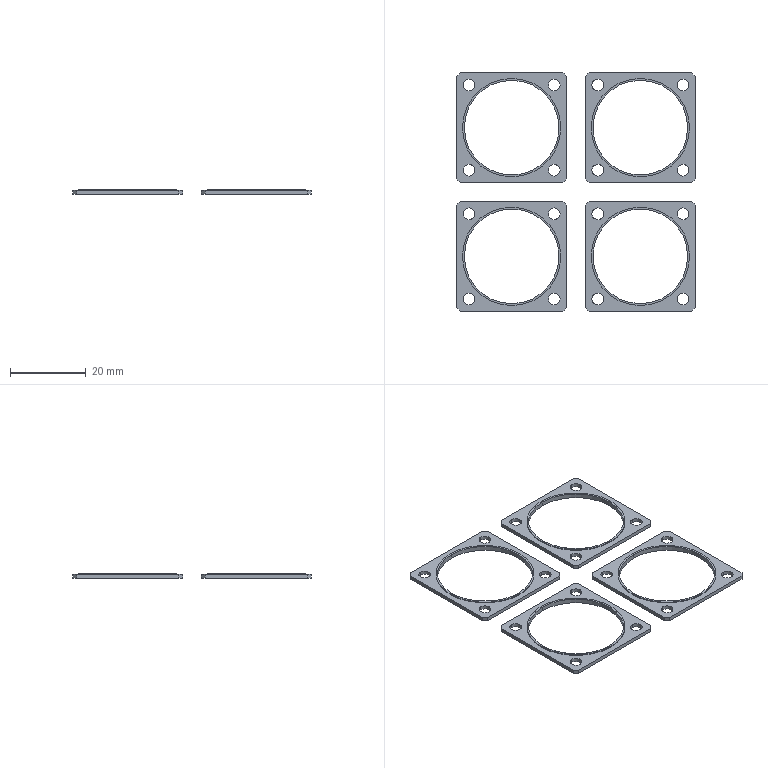CAM job | Mastercam | mm | 9 operations | part box 63 x 63 x 1.2
1. 2D High Speed (2D Area Mill) | 1 - 6C
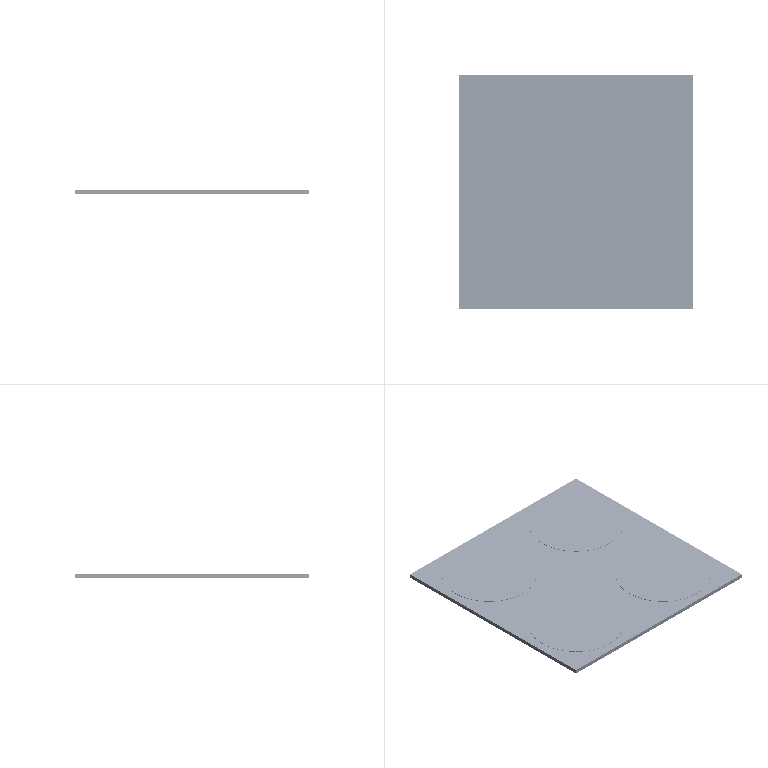2. Contour (Ramp) | 1 - 6C
3. Contour (Ramp) | 3 - 2C
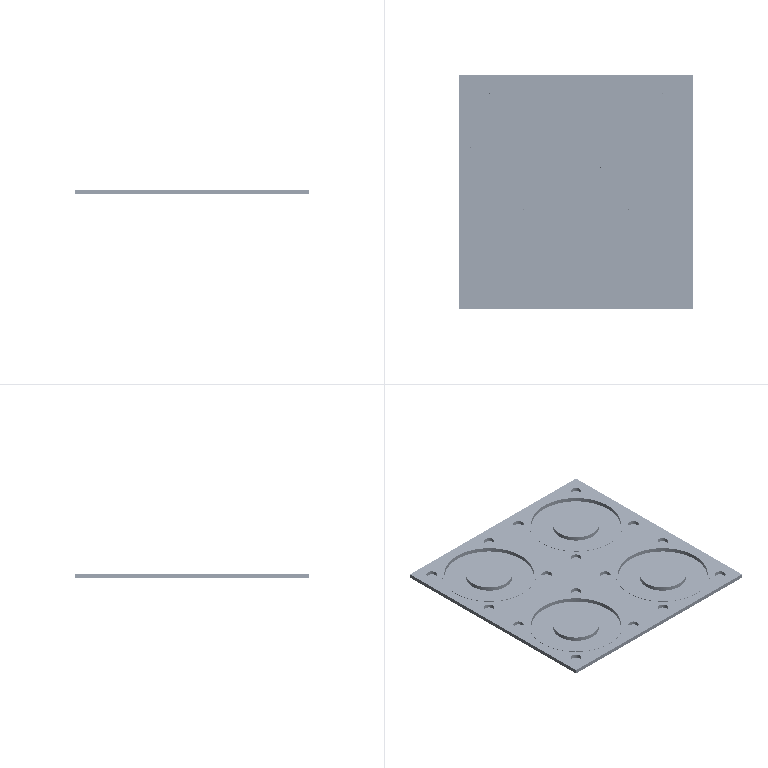4. Contour (2D) | 4 - 2J
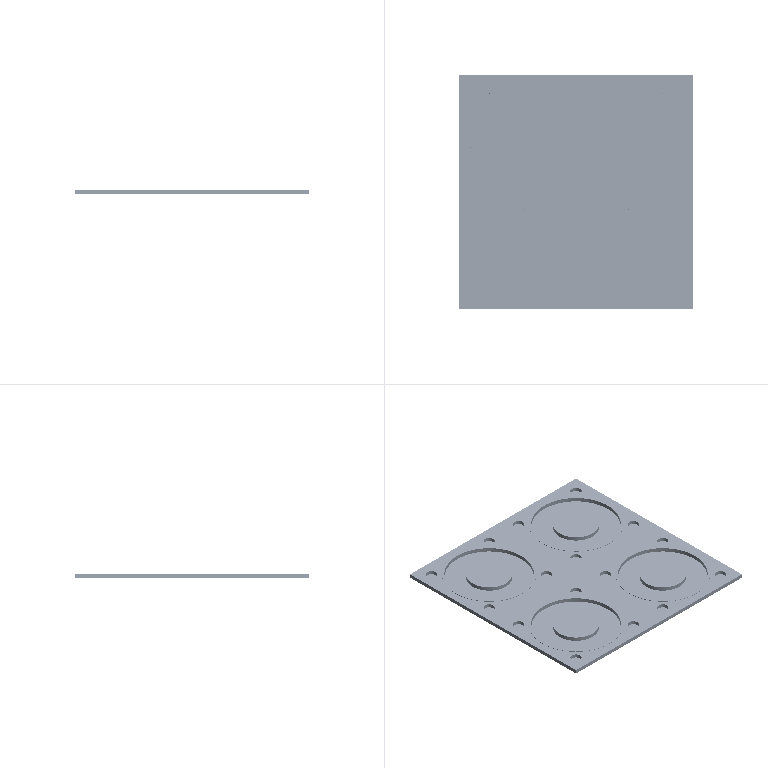5. 2D High Speed (2D Area Mill) | 2 - 6J
6. Contour (2D) | 2 - 6J
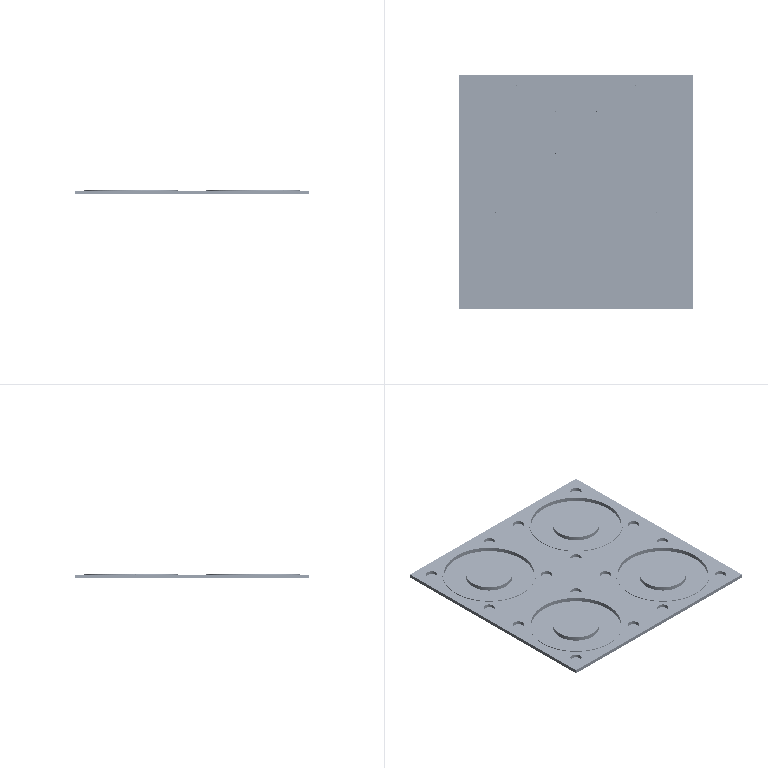7. Model Chamfer | 5 - 4 倒角刀
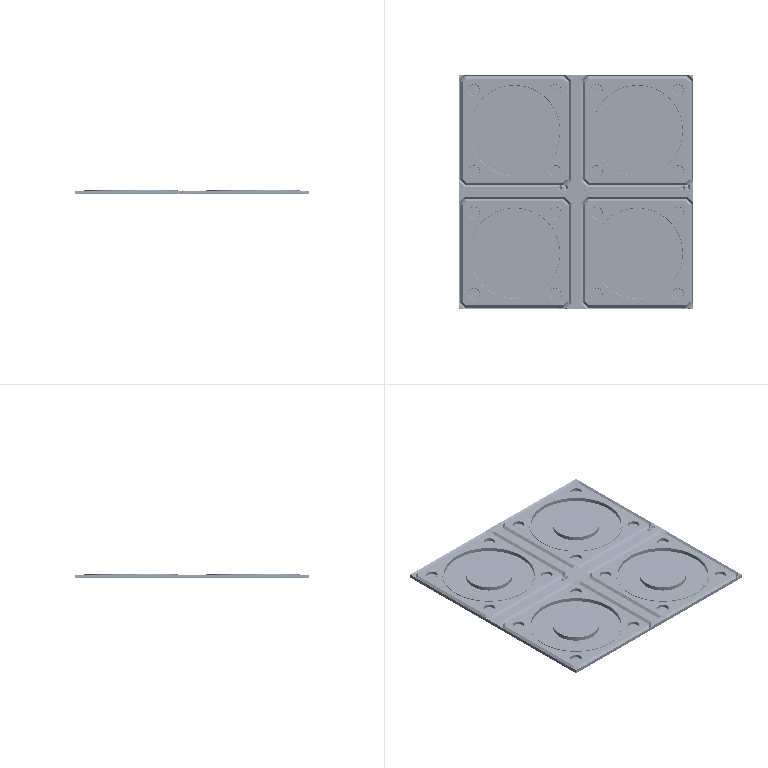8. Contour (Ramp) | 6 - 4C
9. Contour (2D) | 7 - 4J